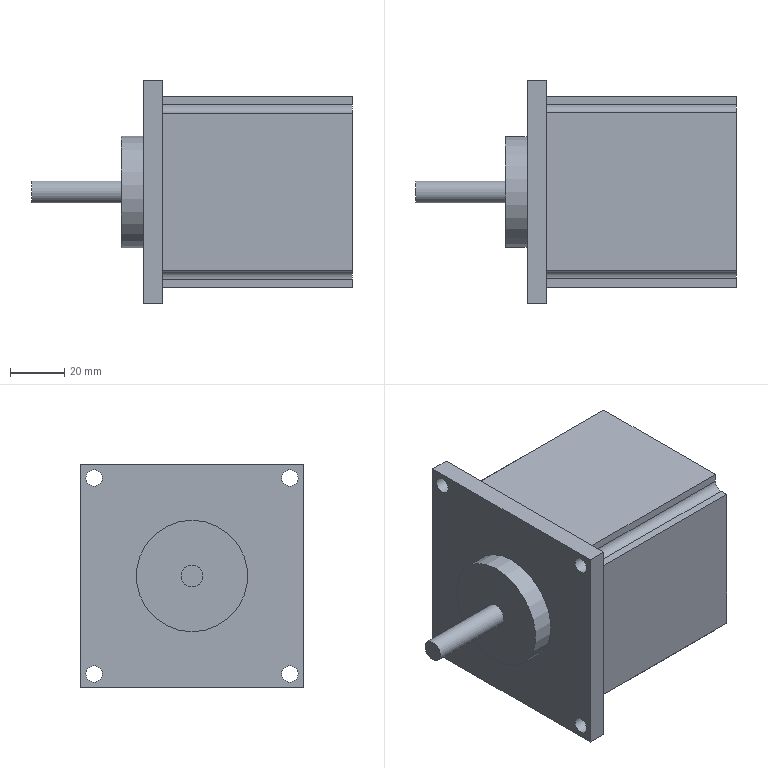Component | NX | MOTOR_2_2 | 1 solid | 31 faces | volume 391958 mm3 | plane 21 | cylinder 10 | commonest cylinder face diameters 6 x8 8 x1 41 x1